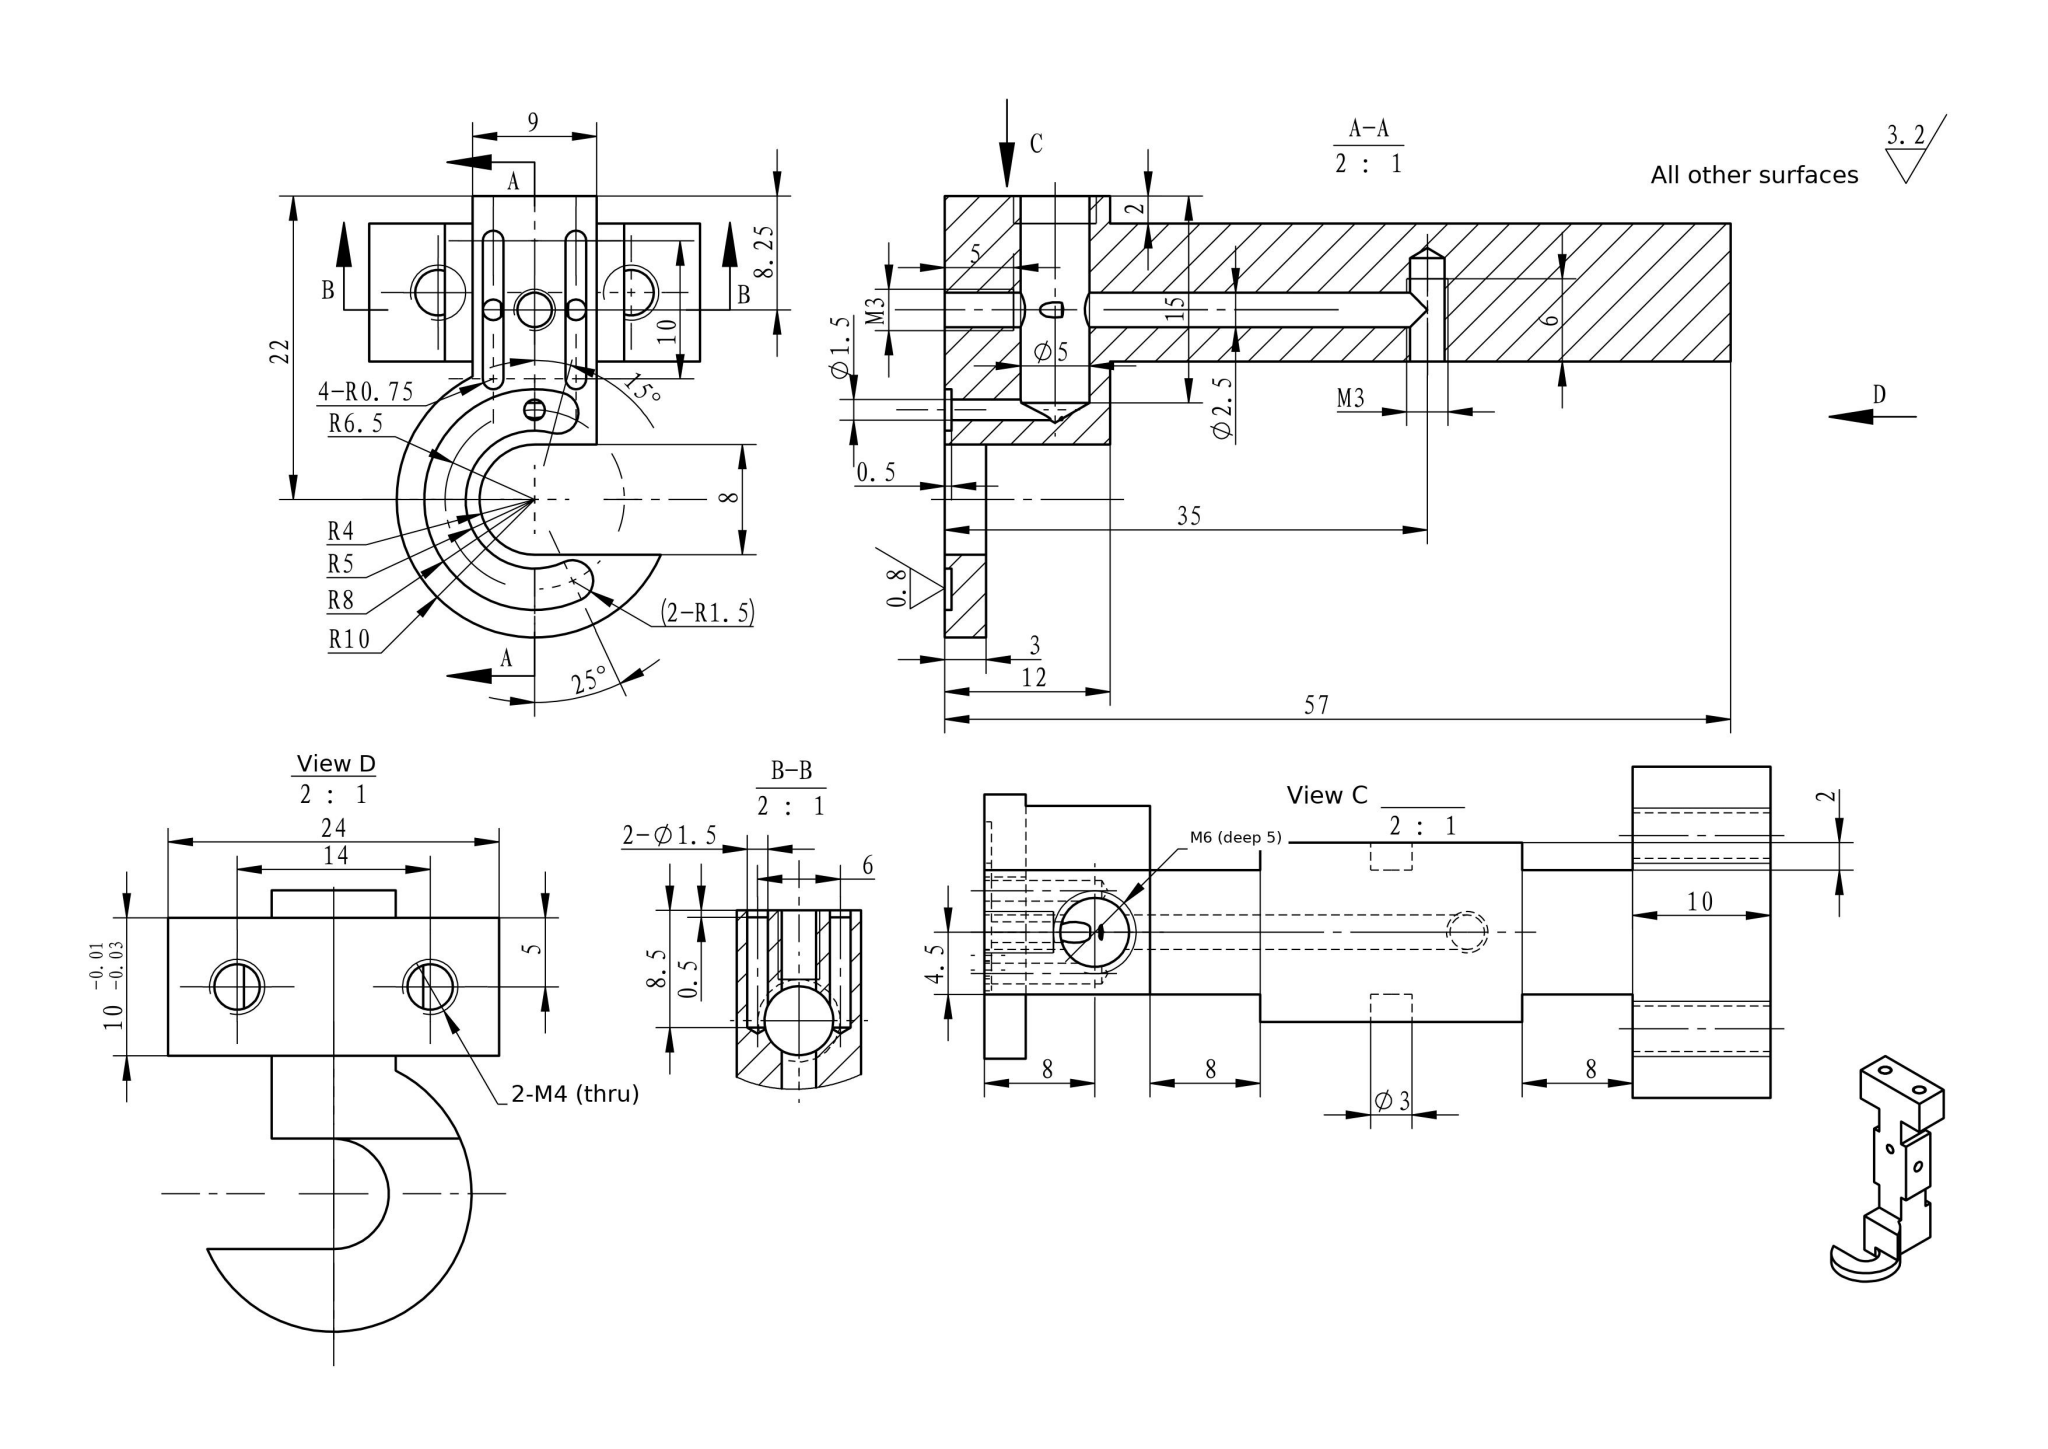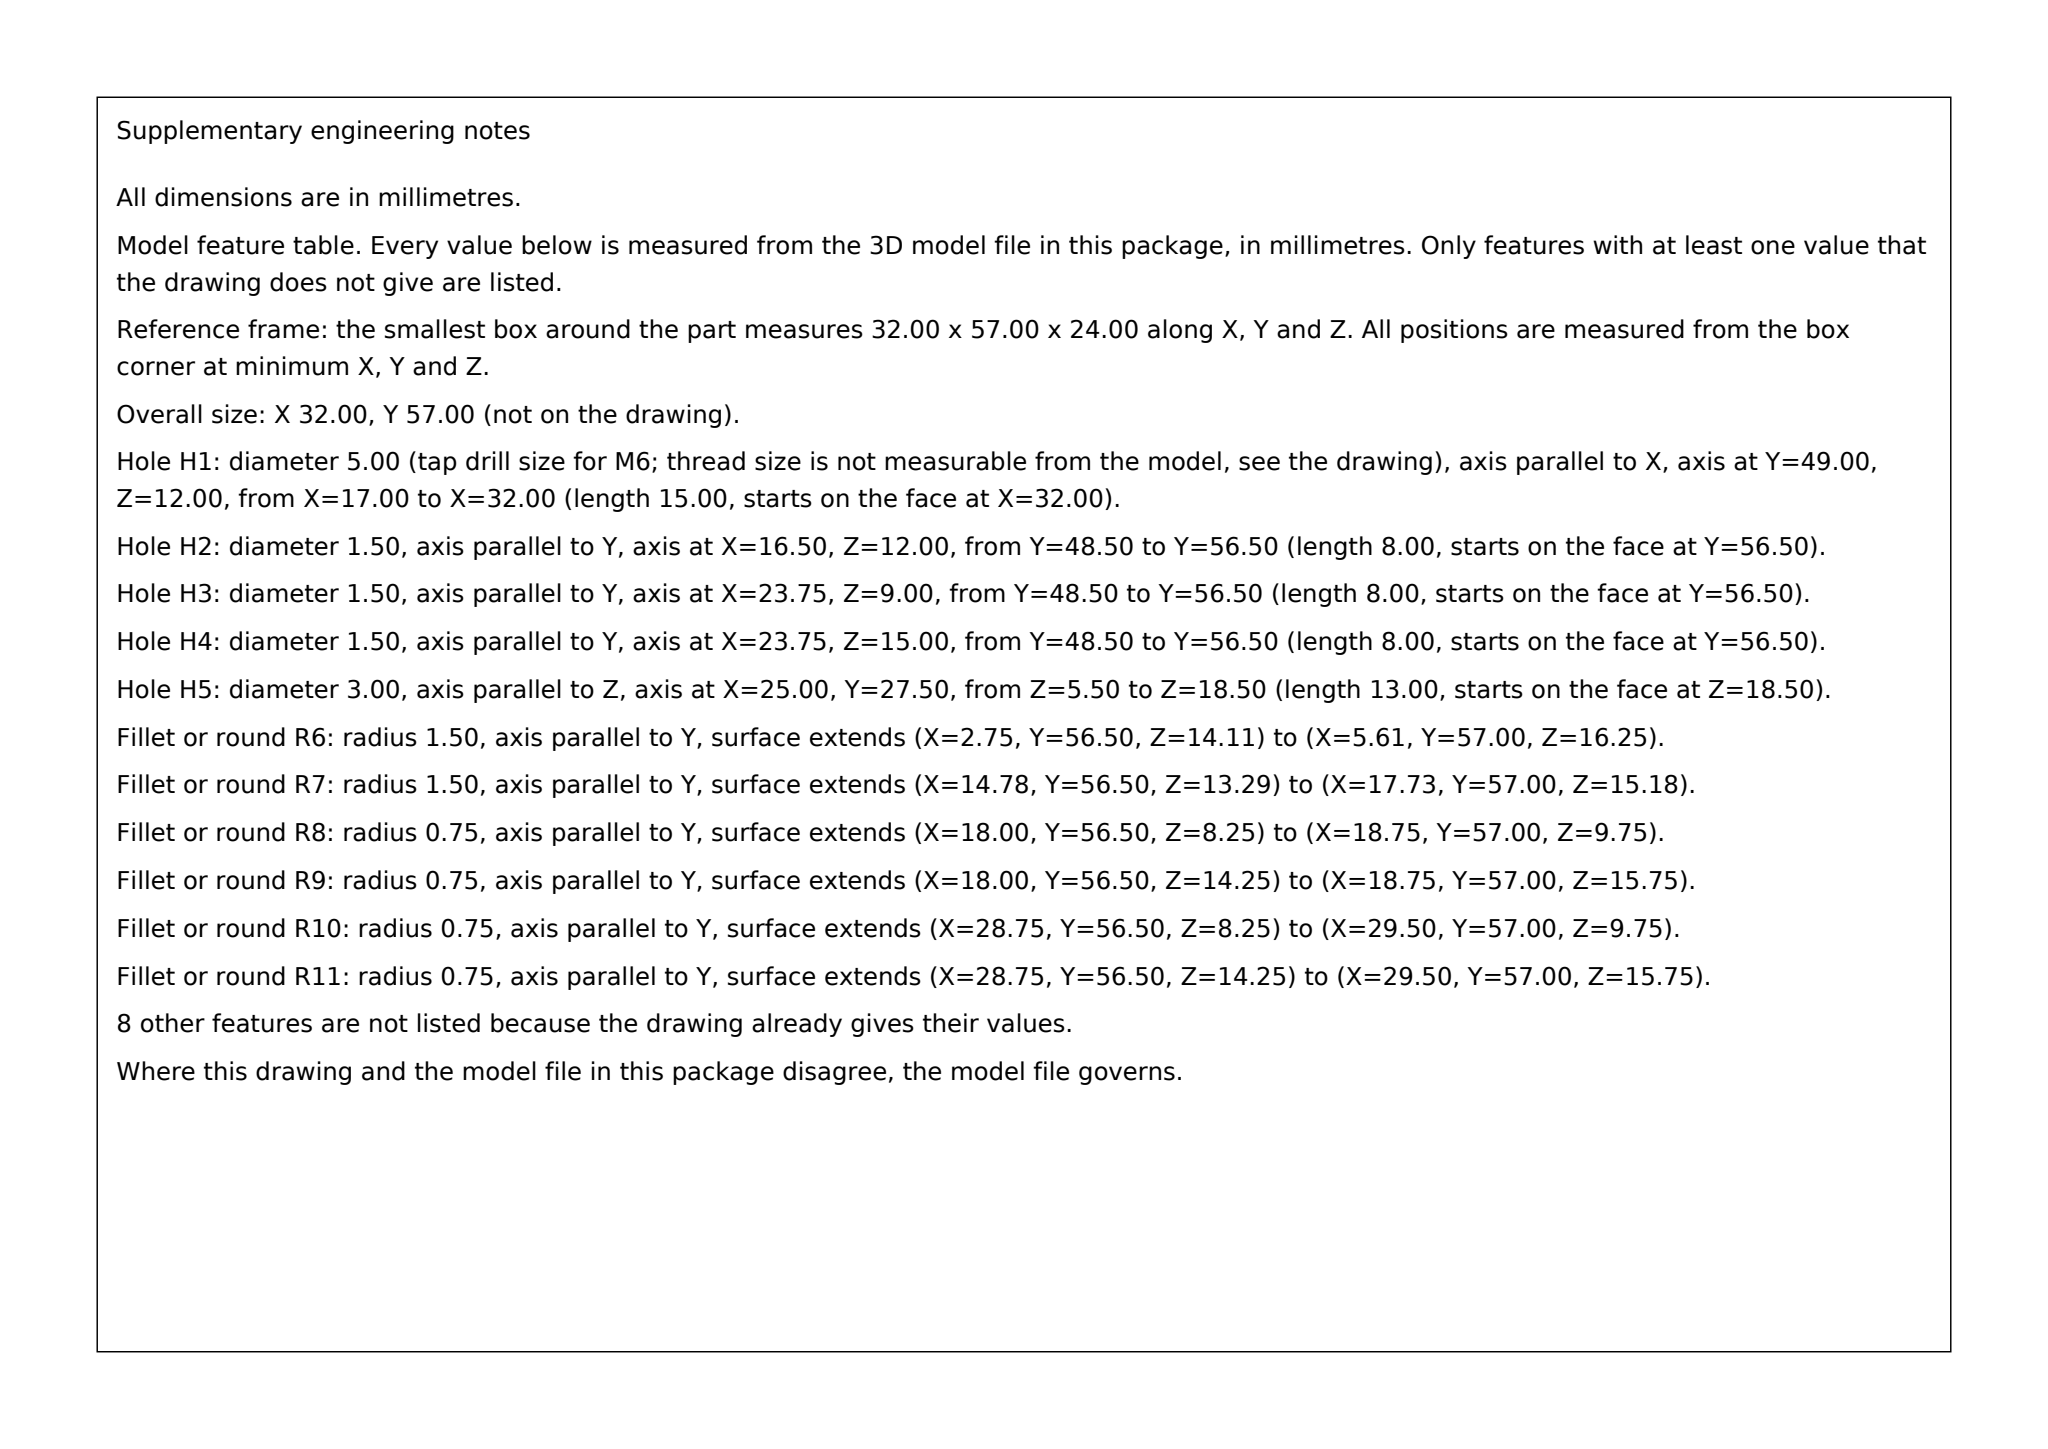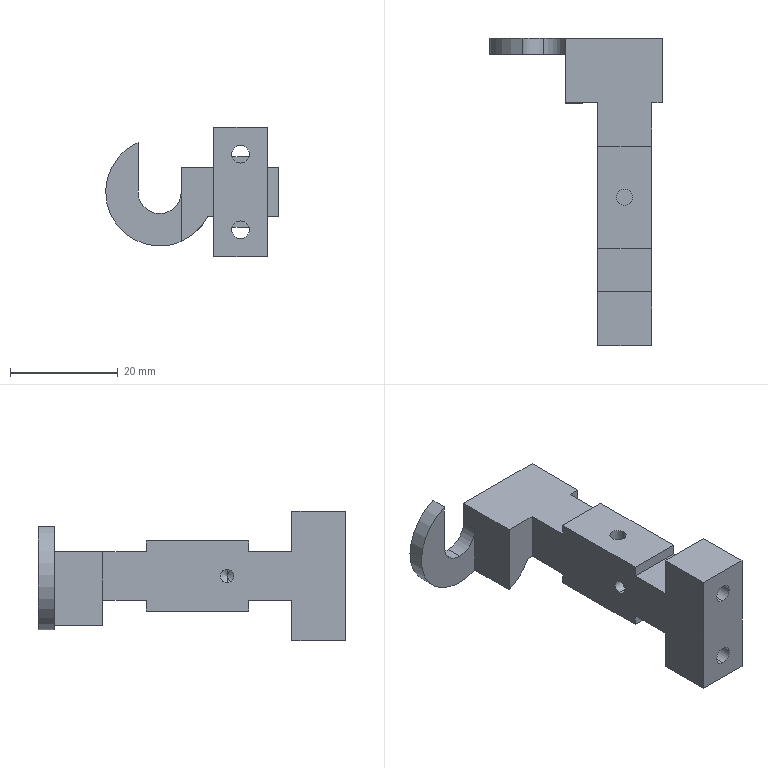Part | SolidWorks | mm | 1 solid | 82 faces | box 32 x 57 x 24 mm | volume 8039 mm3 | cylinder 38 | plane 35 | cone 9 | commonest cylinder face diameters 1.5 x11 2.5 x7 3 x6 3.3 x4 5 x2 16 x2 20 x2 10 x2